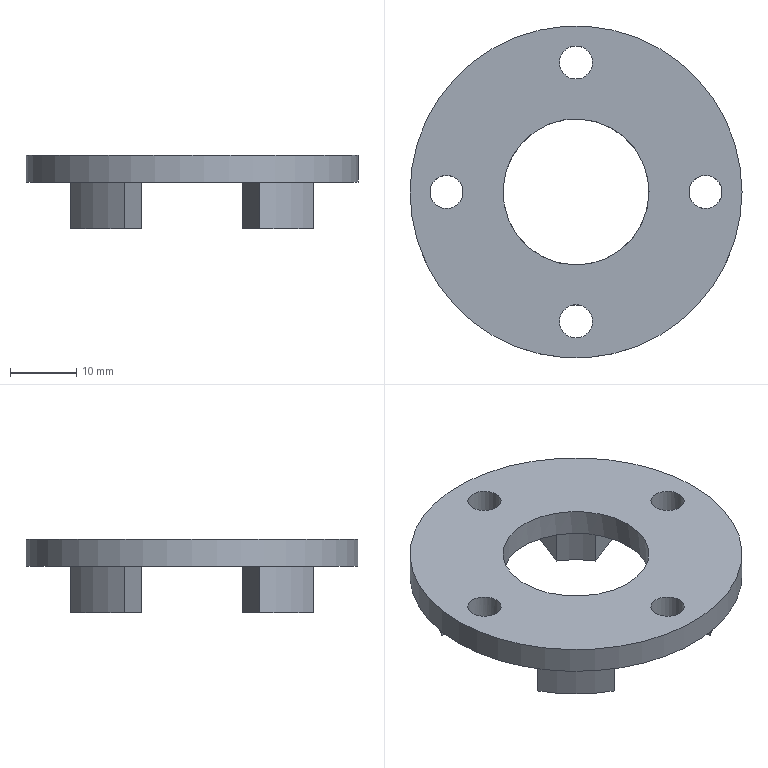Component | NX | COVER | 1 solid | 28 faces | volume 7750 mm3 | plane 14 | cylinder 14 | commonest cylinder face diameters 28 x4 42 x4 5 x4 50 x1 22 x1